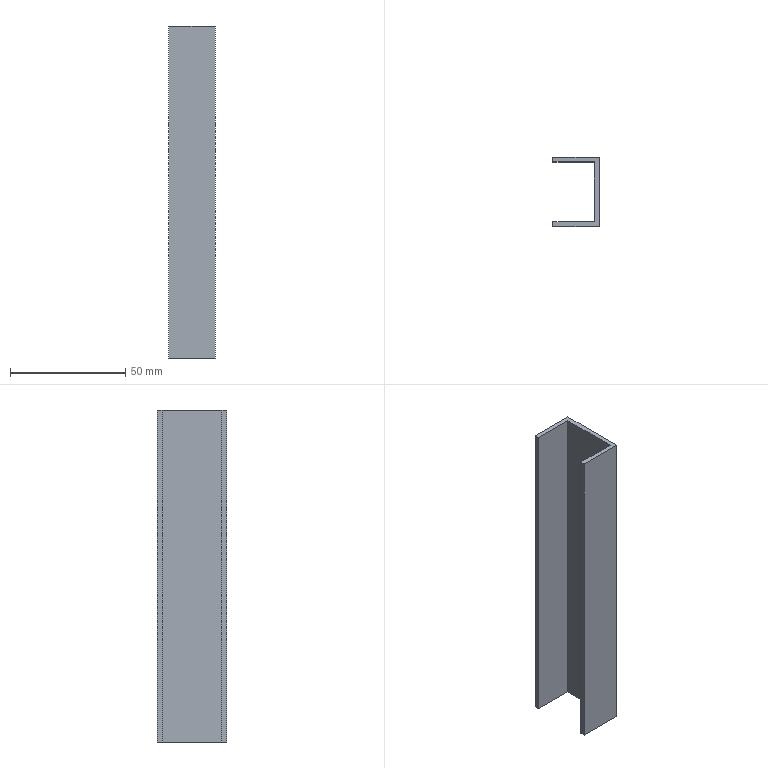Component | SolidWorks | Copy(2)CopyOfPart3-1 | 1 solid | 10 faces | box 20 x 30 x 144 mm | volume 19008 mm3 | plane 10
build123d program:
from build123d import *

# Parameters (mm, degrees)
EXTRUDE_THIN1_DEPTH = 144


with BuildPart() as part:
    # Sketch1 → Extrude-Thin1 (new body)
    with BuildSketch(Plane.XY):
        Polygon((-20, 15.876), (0, 15.876), (0, -14.124), (-20, -14.124), (-20, -12.124), (-2, -12.124), (-2, 13.876), (-20, 13.876), align=None)
    extrude(amount=EXTRUDE_THIN1_DEPTH)


solid = part.part

# Placed as in the assembly
solid = solid.moved(Location((152, 414.124, -488.092), (0, 0, 0)))
STEP:
#1=COLOUR_RGB('',0.7922,0.8196,0.9333);
#2=FILL_AREA_STYLE_COLOUR('',#1);
#3=FILL_AREA_STYLE('',(#2));
#4=SURFACE_STYLE_FILL_AREA(#3);
#5=SURFACE_SIDE_STYLE('',(#4));
#6=SURFACE_STYLE_USAGE(.BOTH.,#5);
#7=PRESENTATION_STYLE_ASSIGNMENT((#6));
#8=CARTESIAN_POINT('',(5.906,15.827,-19.216));
#9=VERTEX_POINT('',#8);
#10=CARTESIAN_POINT('',(5.197,15.827,-19.216));
#11=VERTEX_POINT('',#10);
#12=CARTESIAN_POINT('',(5.984,15.827,-19.216));
#13=DIRECTION('',(-1.,-0.,0.));
#14=VECTOR('',#13,39.37);
#15=LINE('',#12,#14);
#16=EDGE_CURVE('',#9,#11,#15,.T.);
#17=ORIENTED_EDGE('',*,*,#16,.T.);
#18=CARTESIAN_POINT('',(5.197,15.827,-13.547));
#19=VERTEX_POINT('',#18);
#20=CARTESIAN_POINT('',(5.197,15.827,-13.547));
#21=DIRECTION('',(0.,0.,-1.));
#22=VECTOR('',#21,39.37);
#23=LINE('',#20,#22);
#24=EDGE_CURVE('',#19,#11,#23,.T.);
#25=ORIENTED_EDGE('',*,*,#24,.F.);
#26=CARTESIAN_POINT('',(5.906,15.827,-13.547));
#27=VERTEX_POINT('',#26);
#28=CARTESIAN_POINT('',(5.984,15.827,-13.547));
#29=DIRECTION('',(-1.,-0.,0.));
#30=VECTOR('',#29,39.37);
#31=LINE('',#28,#30);
#32=EDGE_CURVE('',#27,#19,#31,.T.);
#33=ORIENTED_EDGE('',*,*,#32,.F.);
#34=CARTESIAN_POINT('',(5.906,15.827,-13.547));
#35=DIRECTION('',(0.,0.,-1.));
#36=VECTOR('',#35,39.37);
#37=LINE('',#34,#36);
#38=EDGE_CURVE('',#27,#9,#37,.T.);
#39=ORIENTED_EDGE('',*,*,#38,.T.);
#40=EDGE_LOOP('',(#17,#25,#33,#39));
#41=FACE_OUTER_BOUND('',#40,.T.);
#42=CARTESIAN_POINT('',(5.984,15.827,-13.547));
#43=DIRECTION('',(0.,-1.,0.));
#44=DIRECTION('',(1.,0.,0.));
#45=AXIS2_PLACEMENT_3D('',#42,#43,#44);
#46=PLANE('',#45);
#47=ADVANCED_FACE('',(#41),#46,.F.);
#48=CARTESIAN_POINT('',(5.197,15.748,-19.216));
#49=VERTEX_POINT('',#48);
#50=CARTESIAN_POINT('',(5.197,15.748,-19.216));
#51=DIRECTION('',(0.,1.,0.));
#52=VECTOR('',#51,39.37);
#53=LINE('',#50,#52);
#54=EDGE_CURVE('',#49,#11,#53,.T.);
#55=ORIENTED_EDGE('',*,*,#54,.F.);
#56=CARTESIAN_POINT('',(5.197,15.748,-13.547));
#57=VERTEX_POINT('',#56);
#58=CARTESIAN_POINT('',(5.197,15.748,-13.547));
#59=DIRECTION('',(0.,0.,-1.));
#60=VECTOR('',#59,39.37);
#61=LINE('',#58,#60);
#62=EDGE_CURVE('',#57,#49,#61,.T.);
#63=ORIENTED_EDGE('',*,*,#62,.F.);
#64=CARTESIAN_POINT('',(5.197,15.748,-13.547));
#65=DIRECTION('',(0.,1.,0.));
#66=VECTOR('',#65,39.37);
#67=LINE('',#64,#66);
#68=EDGE_CURVE('',#57,#19,#67,.T.);
#69=ORIENTED_EDGE('',*,*,#68,.T.);
#70=ORIENTED_EDGE('',*,*,#24,.T.);
#71=EDGE_LOOP('',(#55,#63,#69,#70));
#72=FACE_OUTER_BOUND('',#71,.T.);
#73=CARTESIAN_POINT('',(5.197,15.748,-13.547));
#74=DIRECTION('',(-1.,0.,0.));
#75=DIRECTION('',(0.,0.,1.));
#76=AXIS2_PLACEMENT_3D('',#73,#74,#75);
#77=PLANE('',#76);
#78=ADVANCED_FACE('',(#72),#77,.T.);
#79=CARTESIAN_POINT('',(5.984,15.748,-19.216));
#80=VERTEX_POINT('',#79);
#81=CARTESIAN_POINT('',(5.984,15.748,-19.216));
#82=DIRECTION('',(-1.,-0.,0.));
#83=VECTOR('',#82,39.37);
#84=LINE('',#81,#83);
#85=EDGE_CURVE('',#80,#49,#84,.T.);
#86=ORIENTED_EDGE('',*,*,#85,.F.);
#87=CARTESIAN_POINT('',(5.984,15.748,-13.547));
#88=VERTEX_POINT('',#87);
#89=CARTESIAN_POINT('',(5.984,15.748,-13.547));
#90=DIRECTION('',(0.,0.,-1.));
#91=VECTOR('',#90,39.37);
#92=LINE('',#89,#91);
#93=EDGE_CURVE('',#88,#80,#92,.T.);
#94=ORIENTED_EDGE('',*,*,#93,.F.);
#95=CARTESIAN_POINT('',(5.984,15.748,-13.547));
#96=DIRECTION('',(-1.,-0.,0.));
#97=VECTOR('',#96,39.37);
#98=LINE('',#95,#97);
#99=EDGE_CURVE('',#88,#57,#98,.T.);
#100=ORIENTED_EDGE('',*,*,#99,.T.);
#101=ORIENTED_EDGE('',*,*,#62,.T.);
#102=EDGE_LOOP('',(#86,#94,#100,#101));
#103=FACE_OUTER_BOUND('',#102,.T.);
#104=CARTESIAN_POINT('',(5.984,15.748,-13.547));
#105=DIRECTION('',(0.,-1.,0.));
#106=DIRECTION('',(1.,0.,0.));
#107=AXIS2_PLACEMENT_3D('',#104,#105,#106);
#108=PLANE('',#107);
#109=ADVANCED_FACE('',(#103),#108,.T.);
#110=CARTESIAN_POINT('',(5.984,16.929,-19.216));
#111=VERTEX_POINT('',#110);
#112=CARTESIAN_POINT('',(5.984,15.748,-19.216));
#113=DIRECTION('',(0.,-1.,0.));
#114=VECTOR('',#113,39.37);
#115=LINE('',#112,#114);
#116=EDGE_CURVE('',#111,#80,#115,.T.);
#117=ORIENTED_EDGE('',*,*,#116,.F.);
#118=CARTESIAN_POINT('',(5.984,16.929,-13.547));
#119=VERTEX_POINT('',#118);
#120=CARTESIAN_POINT('',(5.984,16.929,-13.547));
#121=DIRECTION('',(0.,0.,-1.));
#122=VECTOR('',#121,39.37);
#123=LINE('',#120,#122);
#124=EDGE_CURVE('',#119,#111,#123,.T.);
#125=ORIENTED_EDGE('',*,*,#124,.F.);
#126=CARTESIAN_POINT('',(5.984,15.748,-13.547));
#127=DIRECTION('',(0.,-1.,0.));
#128=VECTOR('',#127,39.37);
#129=LINE('',#126,#128);
#130=EDGE_CURVE('',#119,#88,#129,.T.);
#131=ORIENTED_EDGE('',*,*,#130,.T.);
#132=ORIENTED_EDGE('',*,*,#93,.T.);
#133=EDGE_LOOP('',(#117,#125,#131,#132));
#134=FACE_OUTER_BOUND('',#133,.T.);
#135=CARTESIAN_POINT('',(5.984,15.748,-13.547));
#136=DIRECTION('',(1.,0.,0.));
#137=DIRECTION('',(0.,0.,-1.));
#138=AXIS2_PLACEMENT_3D('',#135,#136,#137);
#139=PLANE('',#138);
#140=ADVANCED_FACE('',(#134),#139,.T.);
#141=CARTESIAN_POINT('',(5.197,16.929,-19.216));
#142=VERTEX_POINT('',#141);
#143=CARTESIAN_POINT('',(5.984,16.929,-19.216));
#144=DIRECTION('',(1.,0.,0.));
#145=VECTOR('',#144,39.37);
#146=LINE('',#143,#145);
#147=EDGE_CURVE('',#142,#111,#146,.T.);
#148=ORIENTED_EDGE('',*,*,#147,.F.);
#149=CARTESIAN_POINT('',(5.197,16.929,-13.547));
#150=VERTEX_POINT('',#149);
#151=CARTESIAN_POINT('',(5.197,16.929,-13.547));
#152=DIRECTION('',(0.,0.,-1.));
#153=VECTOR('',#152,39.37);
#154=LINE('',#151,#153);
#155=EDGE_CURVE('',#150,#142,#154,.T.);
#156=ORIENTED_EDGE('',*,*,#155,.F.);
#157=CARTESIAN_POINT('',(5.984,16.929,-13.547));
#158=DIRECTION('',(1.,0.,0.));
#159=VECTOR('',#158,39.37);
#160=LINE('',#157,#159);
#161=EDGE_CURVE('',#150,#119,#160,.T.);
#162=ORIENTED_EDGE('',*,*,#161,.T.);
#163=ORIENTED_EDGE('',*,*,#124,.T.);
#164=EDGE_LOOP('',(#148,#156,#162,#163));
#165=FACE_OUTER_BOUND('',#164,.T.);
#166=CARTESIAN_POINT('',(5.984,16.929,-13.547));
#167=DIRECTION('',(0.,1.,0.));
#168=DIRECTION('',(0.,0.,1.));
#169=AXIS2_PLACEMENT_3D('',#166,#167,#168);
#170=PLANE('',#169);
#171=ADVANCED_FACE('',(#165),#170,.T.);
#172=CARTESIAN_POINT('',(5.197,16.85,-19.216));
#173=VERTEX_POINT('',#172);
#174=CARTESIAN_POINT('',(5.197,16.85,-19.216));
#175=DIRECTION('',(0.,1.,0.));
#176=VECTOR('',#175,39.37);
#177=LINE('',#174,#176);
#178=EDGE_CURVE('',#173,#142,#177,.T.);
#179=ORIENTED_EDGE('',*,*,#178,.F.);
#180=CARTESIAN_POINT('',(5.197,16.85,-13.547));
#181=VERTEX_POINT('',#180);
#182=CARTESIAN_POINT('',(5.197,16.85,-13.547));
#183=DIRECTION('',(0.,0.,-1.));
#184=VECTOR('',#183,39.37);
#185=LINE('',#182,#184);
#186=EDGE_CURVE('',#181,#173,#185,.T.);
#187=ORIENTED_EDGE('',*,*,#186,.F.);
#188=CARTESIAN_POINT('',(5.197,16.85,-13.547));
#189=DIRECTION('',(0.,1.,0.));
#190=VECTOR('',#189,39.37);
#191=LINE('',#188,#190);
#192=EDGE_CURVE('',#181,#150,#191,.T.);
#193=ORIENTED_EDGE('',*,*,#192,.T.);
#194=ORIENTED_EDGE('',*,*,#155,.T.);
#195=EDGE_LOOP('',(#179,#187,#193,#194));
#196=FACE_OUTER_BOUND('',#195,.T.);
#197=CARTESIAN_POINT('',(5.197,16.85,-13.547));
#198=DIRECTION('',(-1.,0.,0.));
#199=DIRECTION('',(0.,0.,1.));
#200=AXIS2_PLACEMENT_3D('',#197,#198,#199);
#201=PLANE('',#200);
#202=ADVANCED_FACE('',(#196),#201,.T.);
#203=CARTESIAN_POINT('',(5.906,16.85,-19.216));
#204=VERTEX_POINT('',#203);
#205=CARTESIAN_POINT('',(5.984,16.85,-19.216));
#206=DIRECTION('',(1.,0.,0.));
#207=VECTOR('',#206,39.37);
#208=LINE('',#205,#207);
#209=EDGE_CURVE('',#173,#204,#208,.T.);
#210=ORIENTED_EDGE('',*,*,#209,.T.);
#211=CARTESIAN_POINT('',(5.906,16.85,-13.547));
#212=VERTEX_POINT('',#211);
#213=CARTESIAN_POINT('',(5.906,16.85,-13.547));
#214=DIRECTION('',(0.,0.,-1.));
#215=VECTOR('',#214,39.37);
#216=LINE('',#213,#215);
#217=EDGE_CURVE('',#212,#204,#216,.T.);
#218=ORIENTED_EDGE('',*,*,#217,.F.);
#219=CARTESIAN_POINT('',(5.984,16.85,-13.547));
#220=DIRECTION('',(1.,0.,0.));
#221=VECTOR('',#220,39.37);
#222=LINE('',#219,#221);
#223=EDGE_CURVE('',#181,#212,#222,.T.);
#224=ORIENTED_EDGE('',*,*,#223,.F.);
#225=ORIENTED_EDGE('',*,*,#186,.T.);
#226=EDGE_LOOP('',(#210,#218,#224,#225));
#227=FACE_OUTER_BOUND('',#226,.T.);
#228=CARTESIAN_POINT('',(5.984,16.85,-13.547));
#229=DIRECTION('',(0.,1.,0.));
#230=DIRECTION('',(0.,0.,1.));
#231=AXIS2_PLACEMENT_3D('',#228,#229,#230);
#232=PLANE('',#231);
#233=ADVANCED_FACE('',(#227),#232,.F.);
#234=CARTESIAN_POINT('',(5.906,15.748,-19.216));
#235=DIRECTION('',(0.,-1.,0.));
#236=VECTOR('',#235,39.37);
#237=LINE('',#234,#236);
#238=EDGE_CURVE('',#204,#9,#237,.T.);
#239=ORIENTED_EDGE('',*,*,#238,.T.);
#240=ORIENTED_EDGE('',*,*,#38,.F.);
#241=CARTESIAN_POINT('',(5.906,15.748,-13.547));
#242=DIRECTION('',(0.,-1.,0.));
#243=VECTOR('',#242,39.37);
#244=LINE('',#241,#243);
#245=EDGE_CURVE('',#212,#27,#244,.T.);
#246=ORIENTED_EDGE('',*,*,#245,.F.);
#247=ORIENTED_EDGE('',*,*,#217,.T.);
#248=EDGE_LOOP('',(#239,#240,#246,#247));
#249=FACE_OUTER_BOUND('',#248,.T.);
#250=CARTESIAN_POINT('',(5.906,15.748,-13.547));
#251=DIRECTION('',(1.,0.,0.));
#252=DIRECTION('',(0.,0.,-1.));
#253=AXIS2_PLACEMENT_3D('',#250,#251,#252);
#254=PLANE('',#253);
#255=ADVANCED_FACE('',(#249),#254,.F.);
#256=ORIENTED_EDGE('',*,*,#32,.T.);
#257=ORIENTED_EDGE('',*,*,#68,.F.);
#258=ORIENTED_EDGE('',*,*,#99,.F.);
#259=ORIENTED_EDGE('',*,*,#130,.F.);
#260=ORIENTED_EDGE('',*,*,#161,.F.);
#261=ORIENTED_EDGE('',*,*,#192,.F.);
#262=ORIENTED_EDGE('',*,*,#223,.T.);
#263=ORIENTED_EDGE('',*,*,#245,.T.);
#264=EDGE_LOOP('',(#256,#257,#258,#259,#260,#261,#262,#263));
#265=FACE_OUTER_BOUND('',#264,.T.);
#266=CARTESIAN_POINT('',(5.984,16.304,-13.547));
#267=DIRECTION('',(0.,0.,-1.));
#268=DIRECTION('',(-1.,0.,0.));
#269=AXIS2_PLACEMENT_3D('',#266,#267,#268);
#270=PLANE('',#269);
#271=ADVANCED_FACE('',(#265),#270,.F.);
#272=ORIENTED_EDGE('',*,*,#16,.F.);
#273=ORIENTED_EDGE('',*,*,#238,.F.);
#274=ORIENTED_EDGE('',*,*,#209,.F.);
#275=ORIENTED_EDGE('',*,*,#178,.T.);
#276=ORIENTED_EDGE('',*,*,#147,.T.);
#277=ORIENTED_EDGE('',*,*,#116,.T.);
#278=ORIENTED_EDGE('',*,*,#85,.T.);
#279=ORIENTED_EDGE('',*,*,#54,.T.);
#280=EDGE_LOOP('',(#272,#273,#274,#275,#276,#277,#278,#279));
#281=FACE_OUTER_BOUND('',#280,.T.);
#282=CARTESIAN_POINT('',(5.984,16.304,-19.216));
#283=DIRECTION('',(0.,0.,-1.));
#284=DIRECTION('',(-1.,0.,0.));
#285=AXIS2_PLACEMENT_3D('',#282,#283,#284);
#286=PLANE('',#285);
#287=ADVANCED_FACE('',(#281),#286,.T.);
#288=CLOSED_SHELL('',(#47,#78,#109,#140,#171,#202,#233,#255,#271,#287));
#289=MANIFOLD_SOLID_BREP('',#288);
#290=STYLED_ITEM('',(#7),#289);
#291=(LENGTH_UNIT()NAMED_UNIT(*)SI_UNIT($,.METRE.));
#292=LENGTH_MEASURE_WITH_UNIT(LENGTH_MEASURE(0.0254),#291);
#293=DIMENSIONAL_EXPONENTS(1.,0.,0.,0.,0.,0.,0.);
#294=(CONVERSION_BASED_UNIT('',#292)LENGTH_UNIT()NAMED_UNIT(#293));
#295=UNCERTAINTY_MEASURE_WITH_UNIT(LENGTH_MEASURE(0.00001),#294,'','');
#296=(NAMED_UNIT(*)PLANE_ANGLE_UNIT()SI_UNIT($,.RADIAN.));
#297=(NAMED_UNIT(*)SI_UNIT($,.STERADIAN.)SOLID_ANGLE_UNIT());
#298=(GEOMETRIC_REPRESENTATION_CONTEXT(3)GLOBAL_UNCERTAINTY_ASSIGNED_CONTEXT((#295))GLOBAL_UNIT_ASSIGNED_CONTEXT((#294,#296,#297))REPRESENTATION_CONTEXT('',''));
#299=MECHANICAL_DESIGN_GEOMETRIC_PRESENTATION_REPRESENTATION('',(#290),#298);
#300=PRESENTATION_LAYER_ASSIGNMENT('','',(#290));
#301=CARTESIAN_POINT('',(0.,0.,0.));
#302=DIRECTION('',(0.,0.,1.));
#303=DIRECTION('',(1.,0.,0.));
#304=AXIS2_PLACEMENT_3D('',#301,#302,#303);
#305=(LENGTH_UNIT()NAMED_UNIT(*)SI_UNIT($,.METRE.));
#306=LENGTH_MEASURE_WITH_UNIT(LENGTH_MEASURE(0.0254),#305);
#307=DIMENSIONAL_EXPONENTS(1.,0.,0.,0.,0.,0.,0.);
#308=(CONVERSION_BASED_UNIT('',#306)LENGTH_UNIT()NAMED_UNIT(#307));
#309=UNCERTAINTY_MEASURE_WITH_UNIT(LENGTH_MEASURE(0.00001),#308,'','');
#310=(NAMED_UNIT(*)PLANE_ANGLE_UNIT()SI_UNIT($,.RADIAN.));
#311=(NAMED_UNIT(*)SI_UNIT($,.STERADIAN.)SOLID_ANGLE_UNIT());
#312=(GEOMETRIC_REPRESENTATION_CONTEXT(3)GLOBAL_UNCERTAINTY_ASSIGNED_CONTEXT((#309))GLOBAL_UNIT_ASSIGNED_CONTEXT((#308,#310,#311))REPRESENTATION_CONTEXT('',''));
#313=ADVANCED_BREP_SHAPE_REPRESENTATION('',(#289,#304),#312);